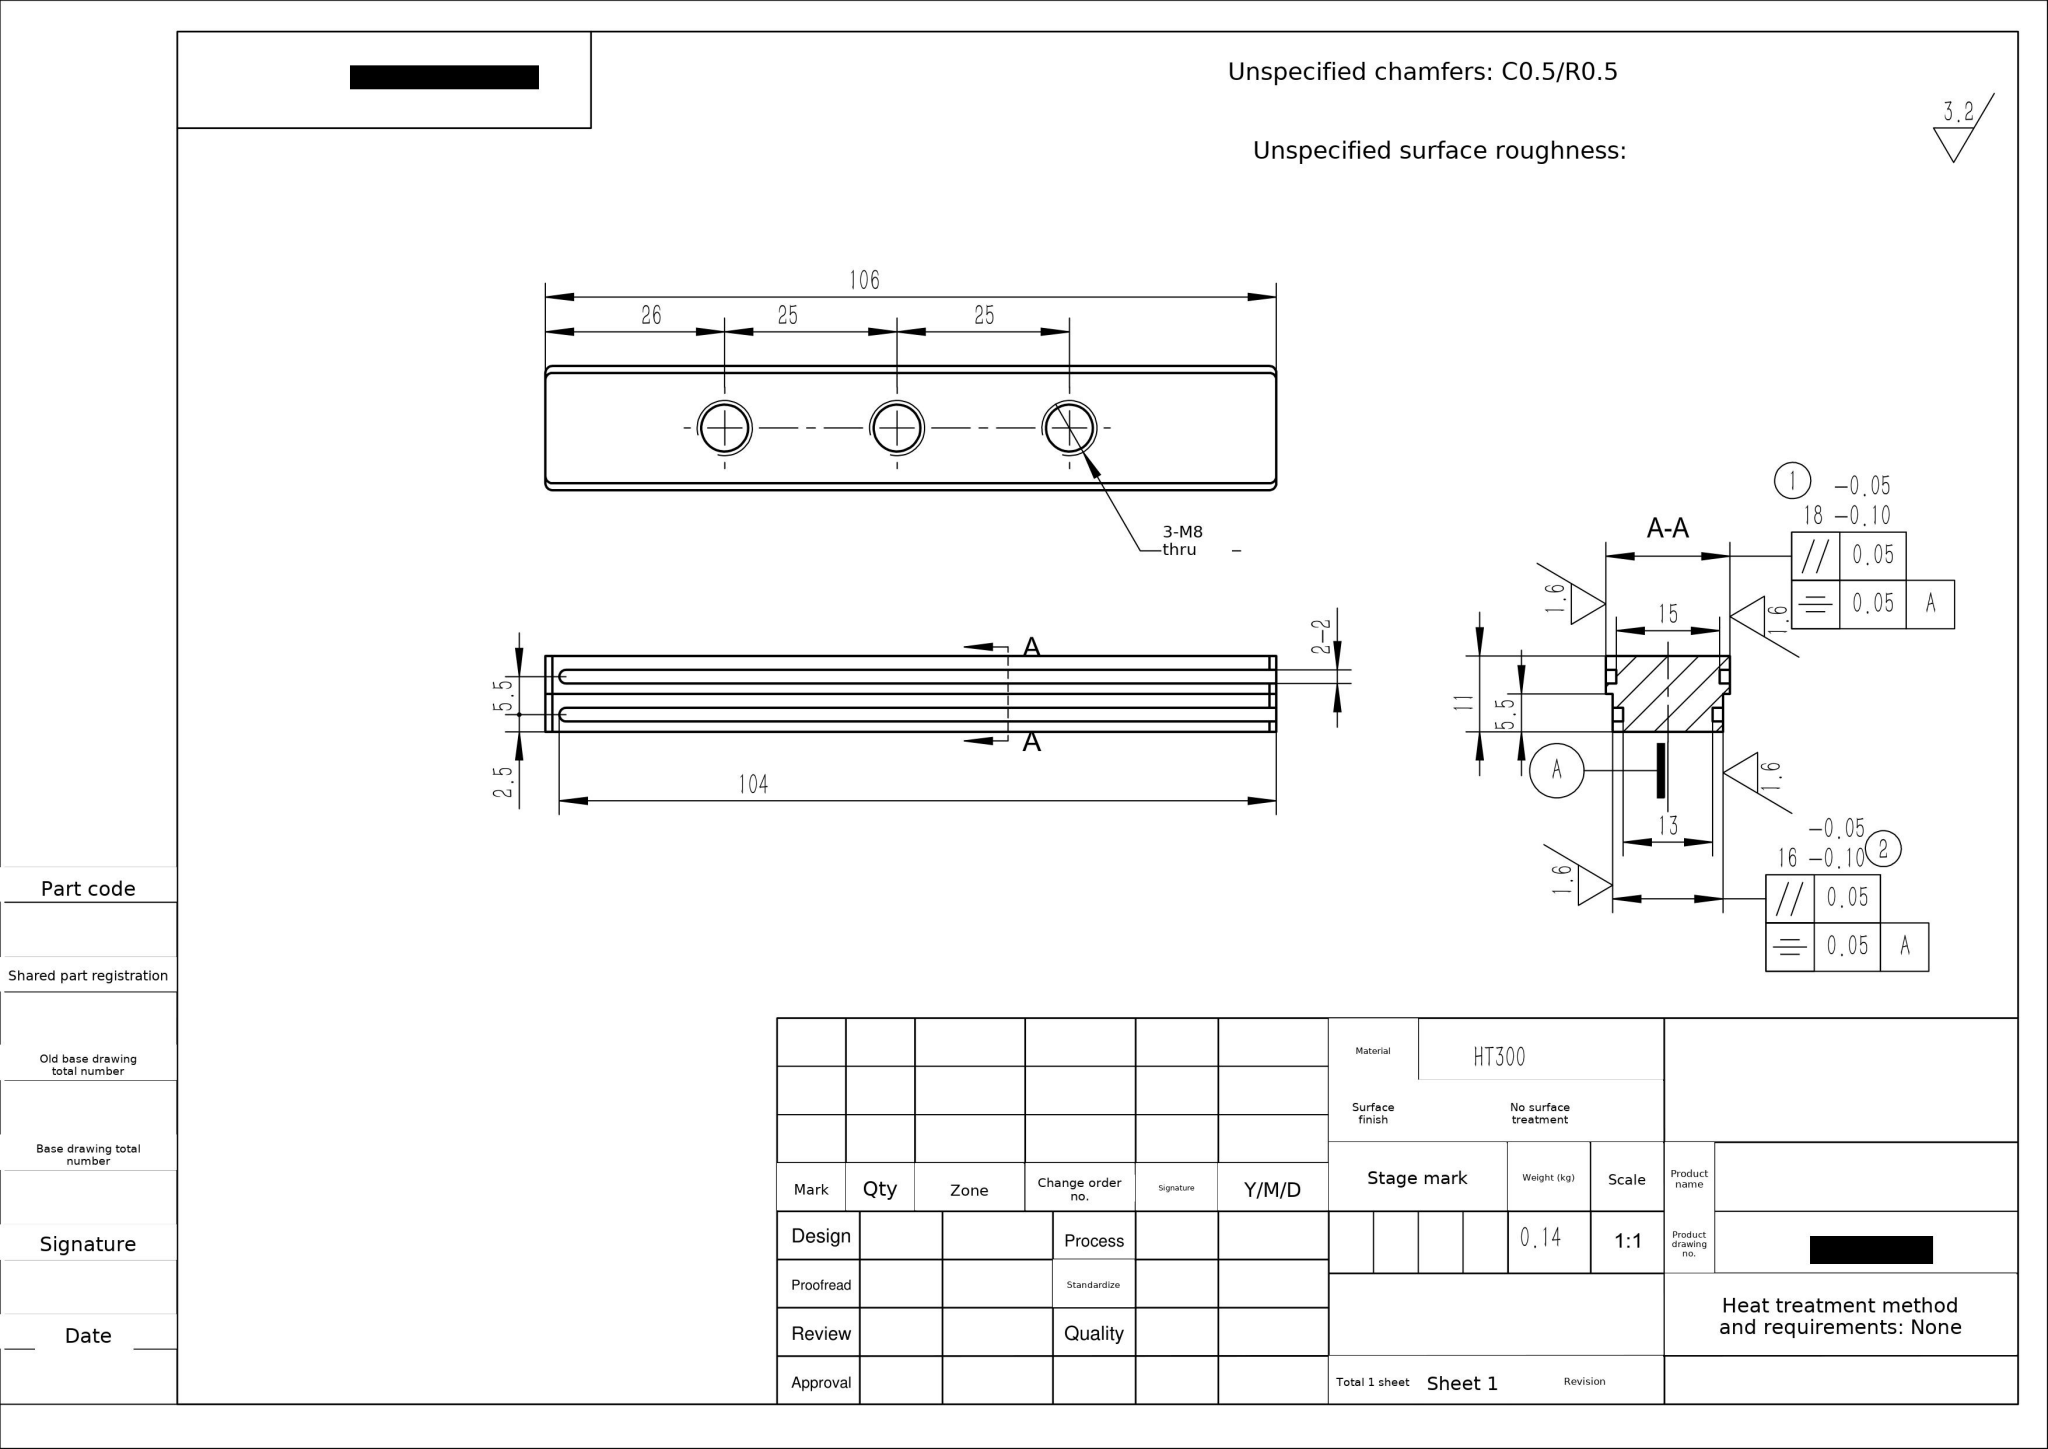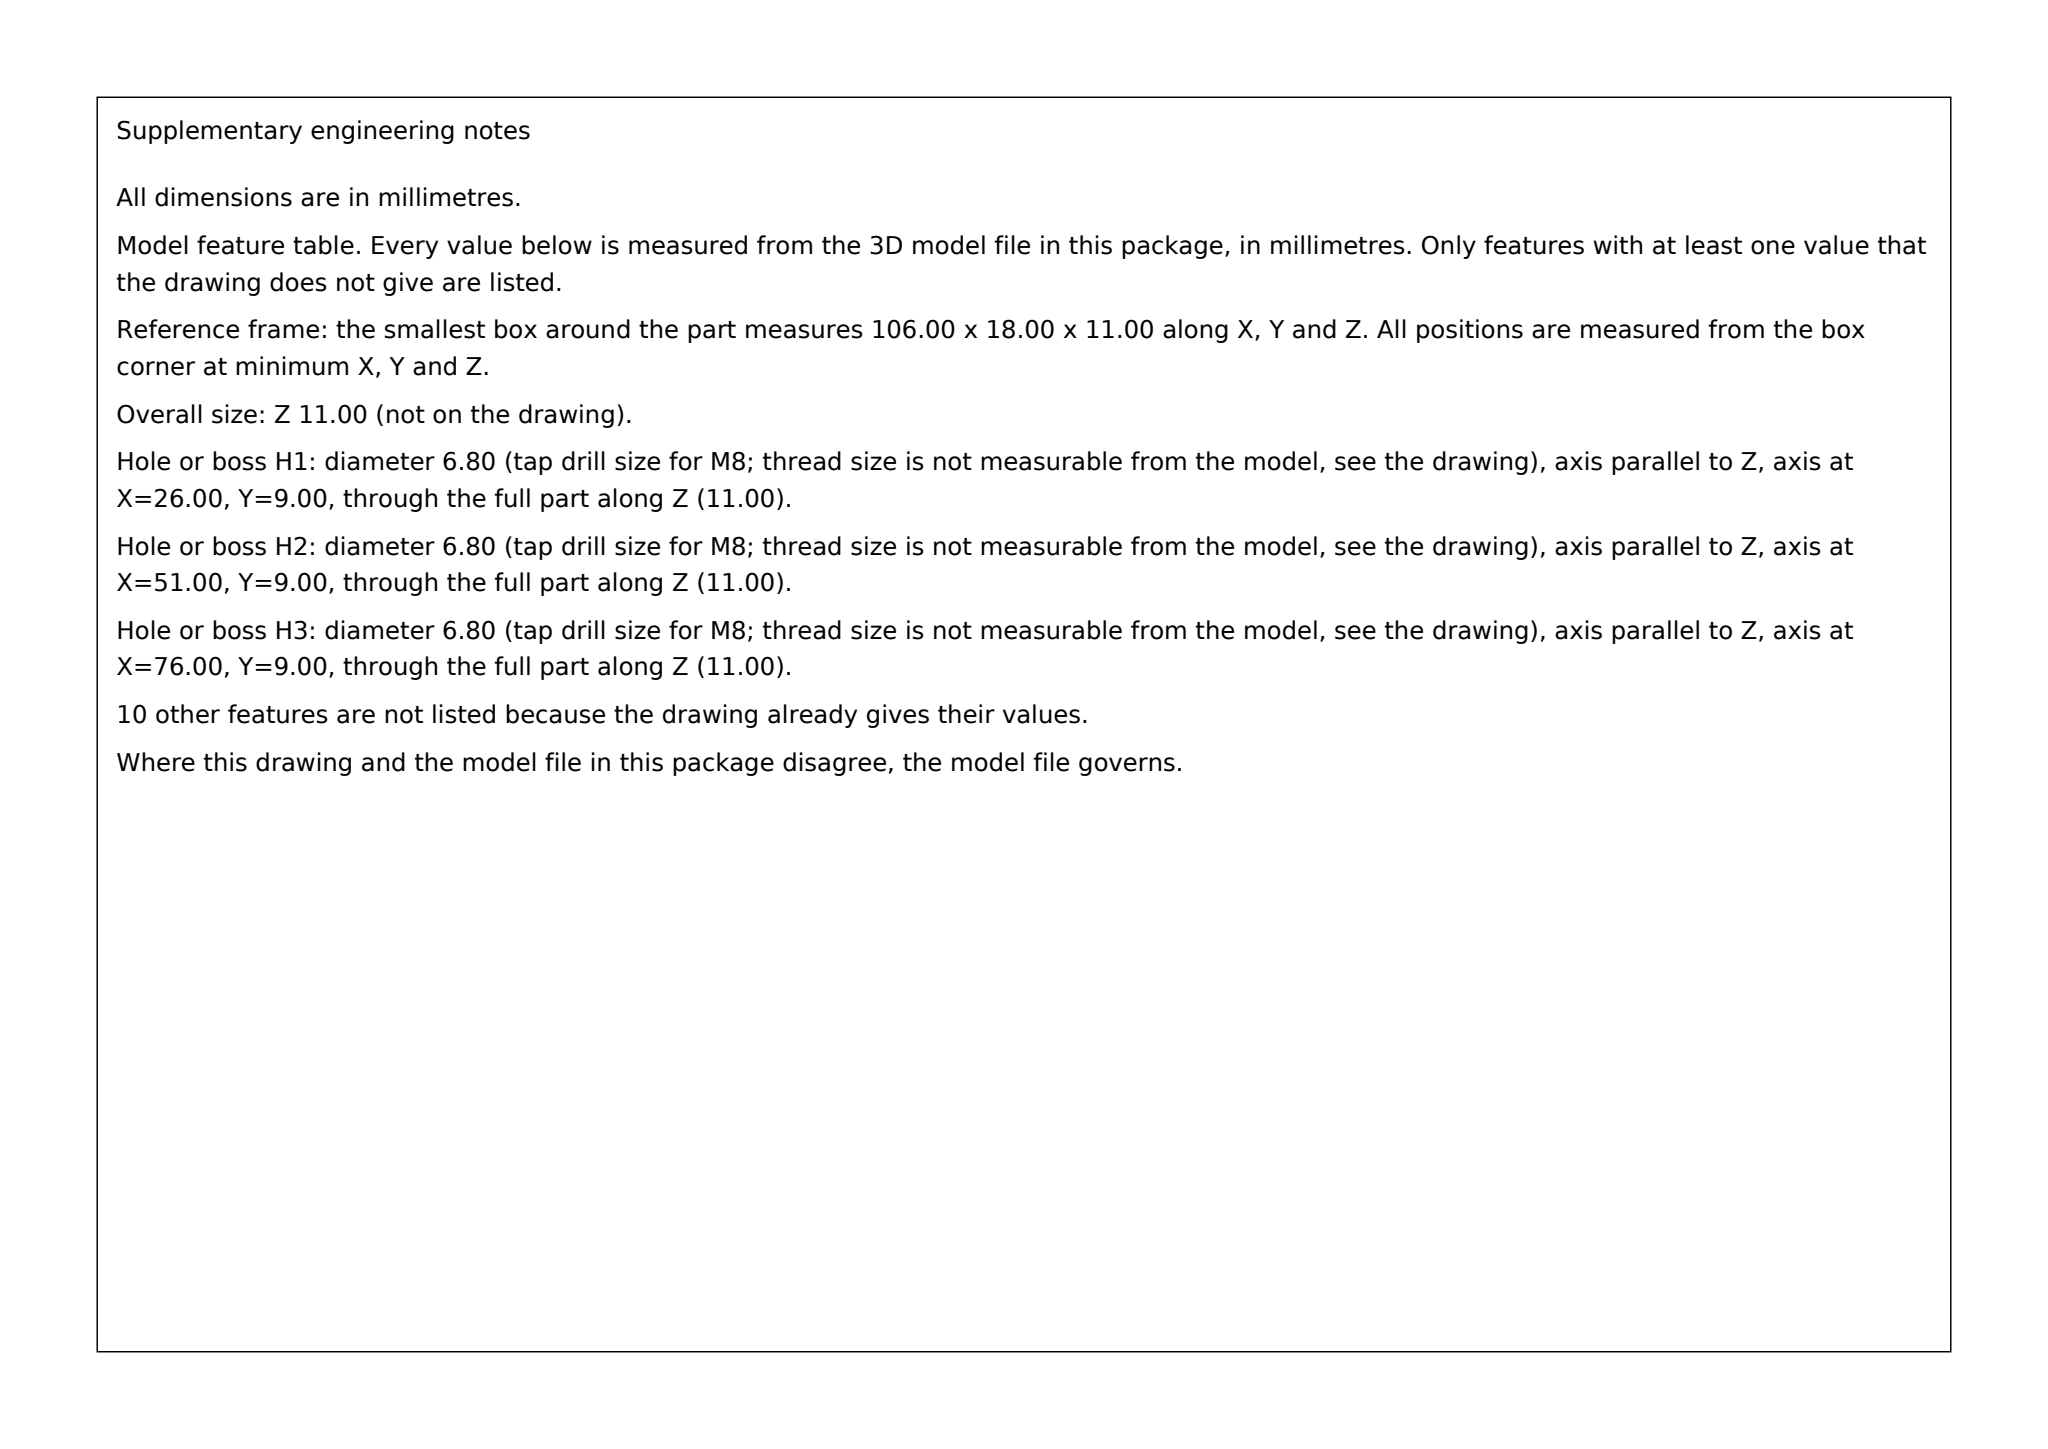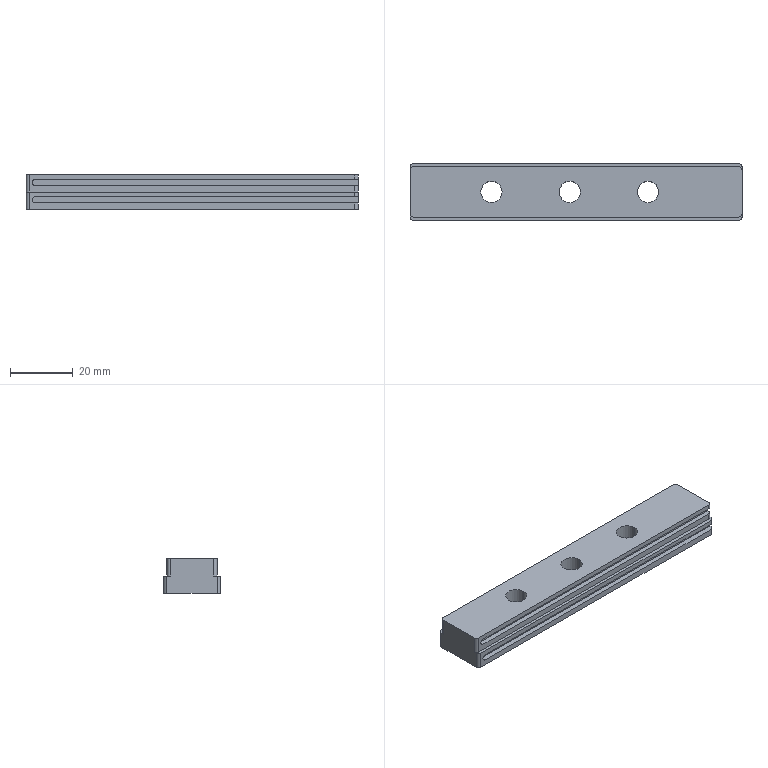Part | SolidWorks | mm | material HT300 | 1 solid | 44 faces | box 106 x 18 x 11 mm | volume 17370 mm3 | cylinder 22 | plane 22 | commonest cylinder face diameters 2 x16 6.8 x6